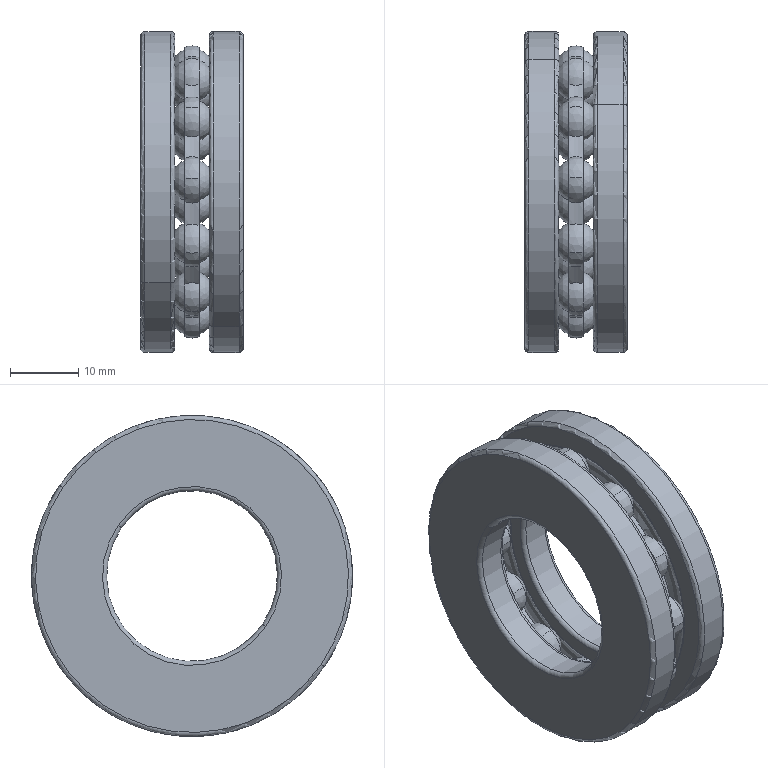Component | SolidWorks | 4-12-12ClampingAxisAssembly-1_4-12-551205Bearing-1 | 15 solids | 164 faces | volume 13454 mm3 | sphere 96 | cylinder 32 | torus 28 | plane 8 | commonest cylinder face diameters 38.083 x12 33.917 x12 47 x4 27 x2 25 x2